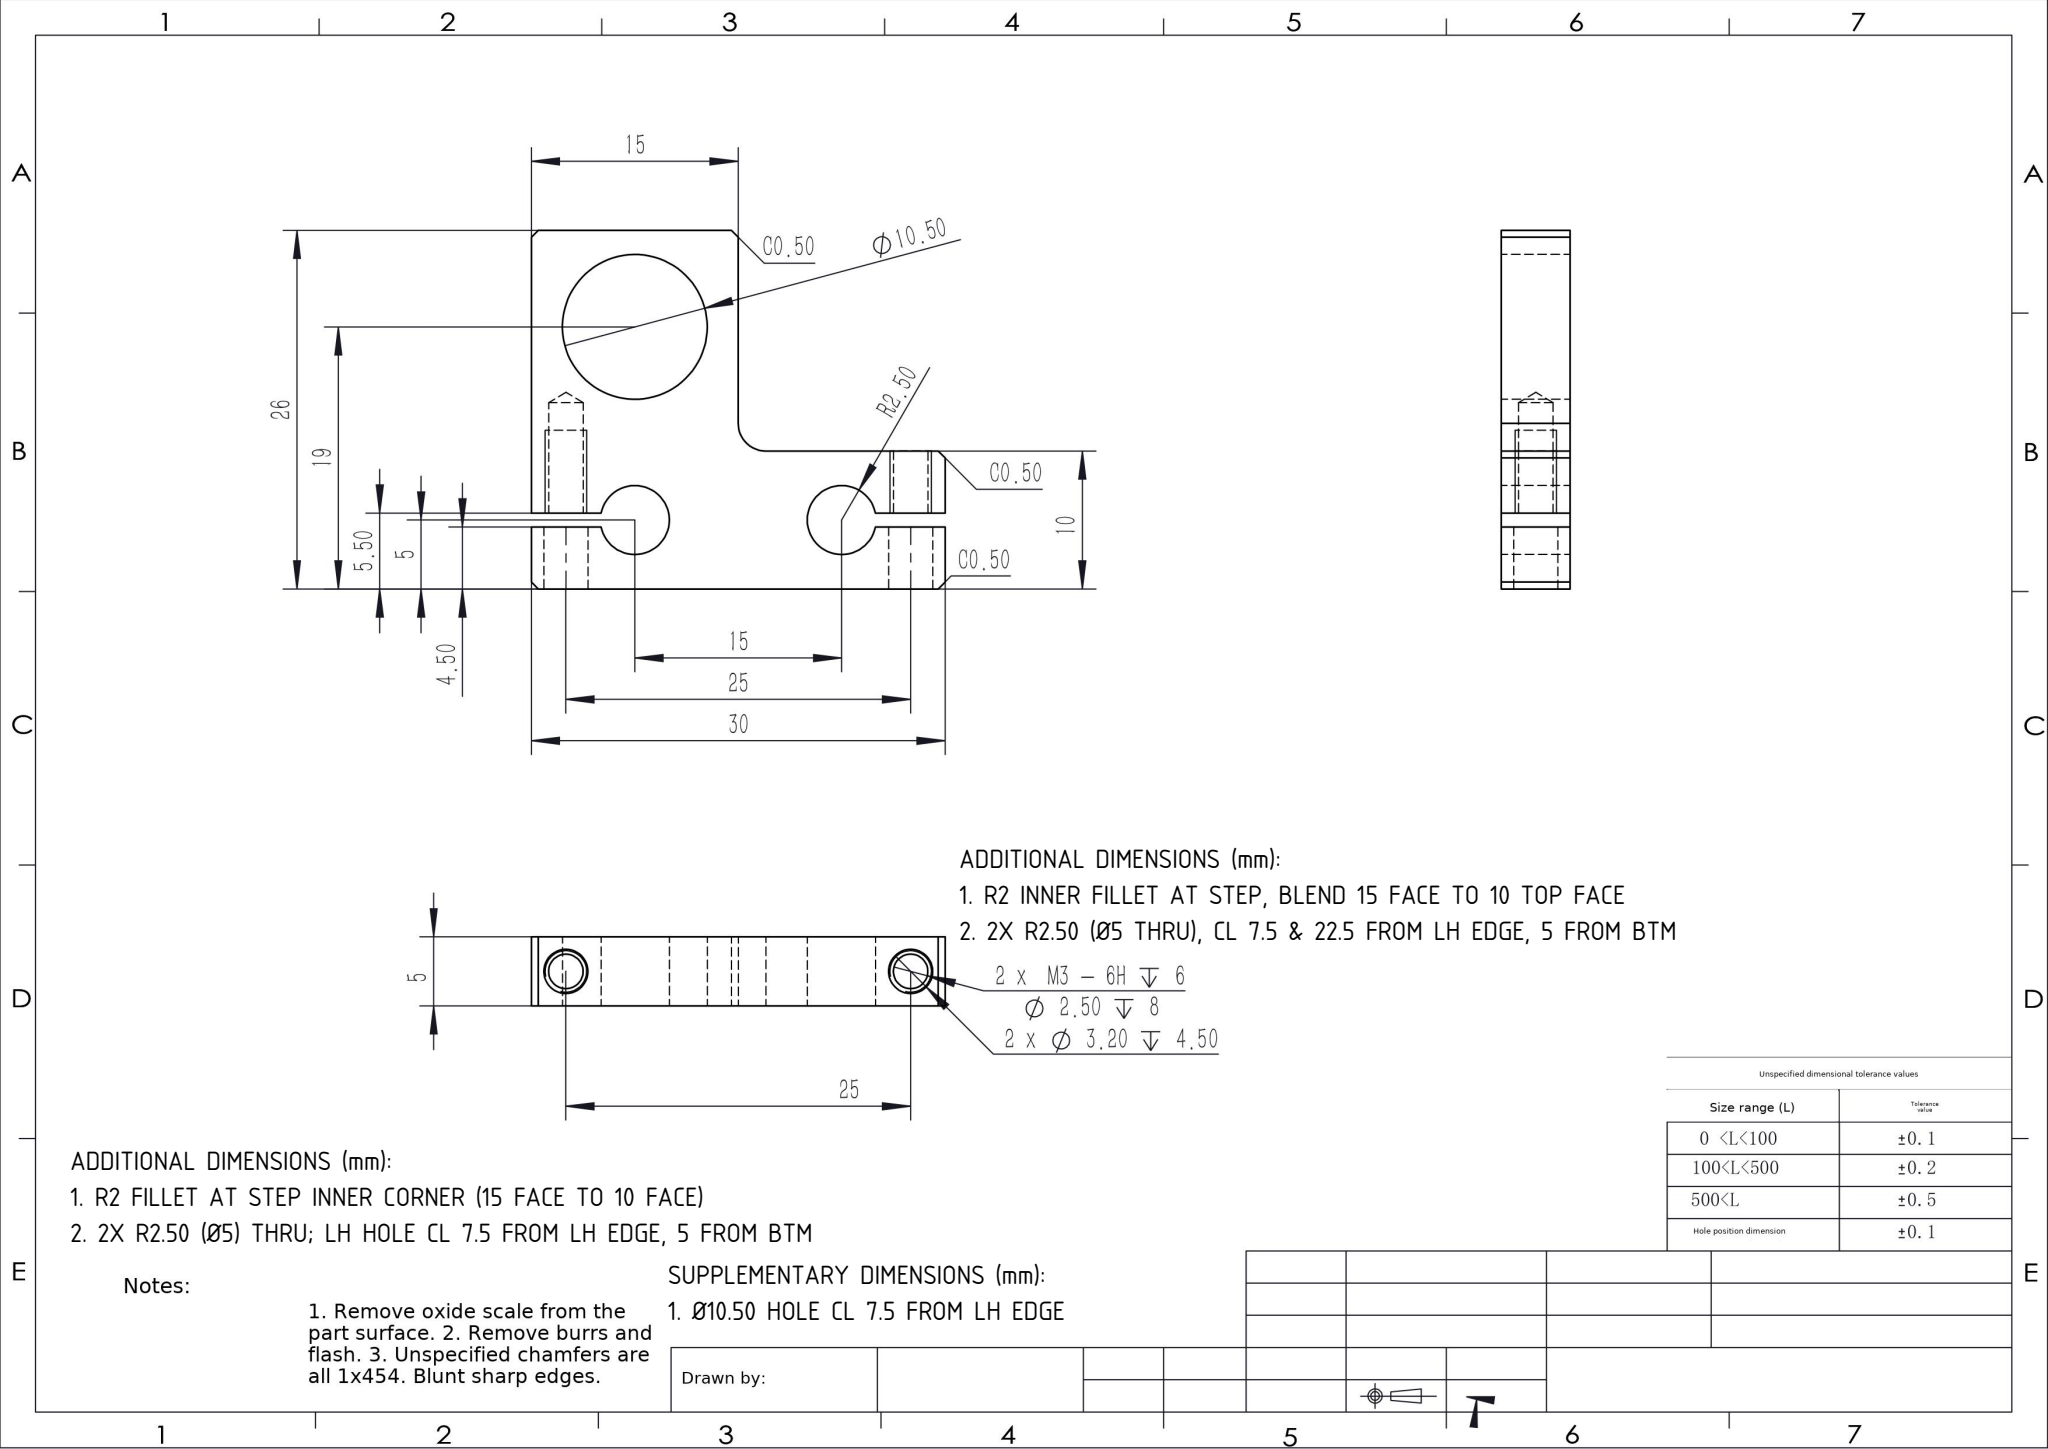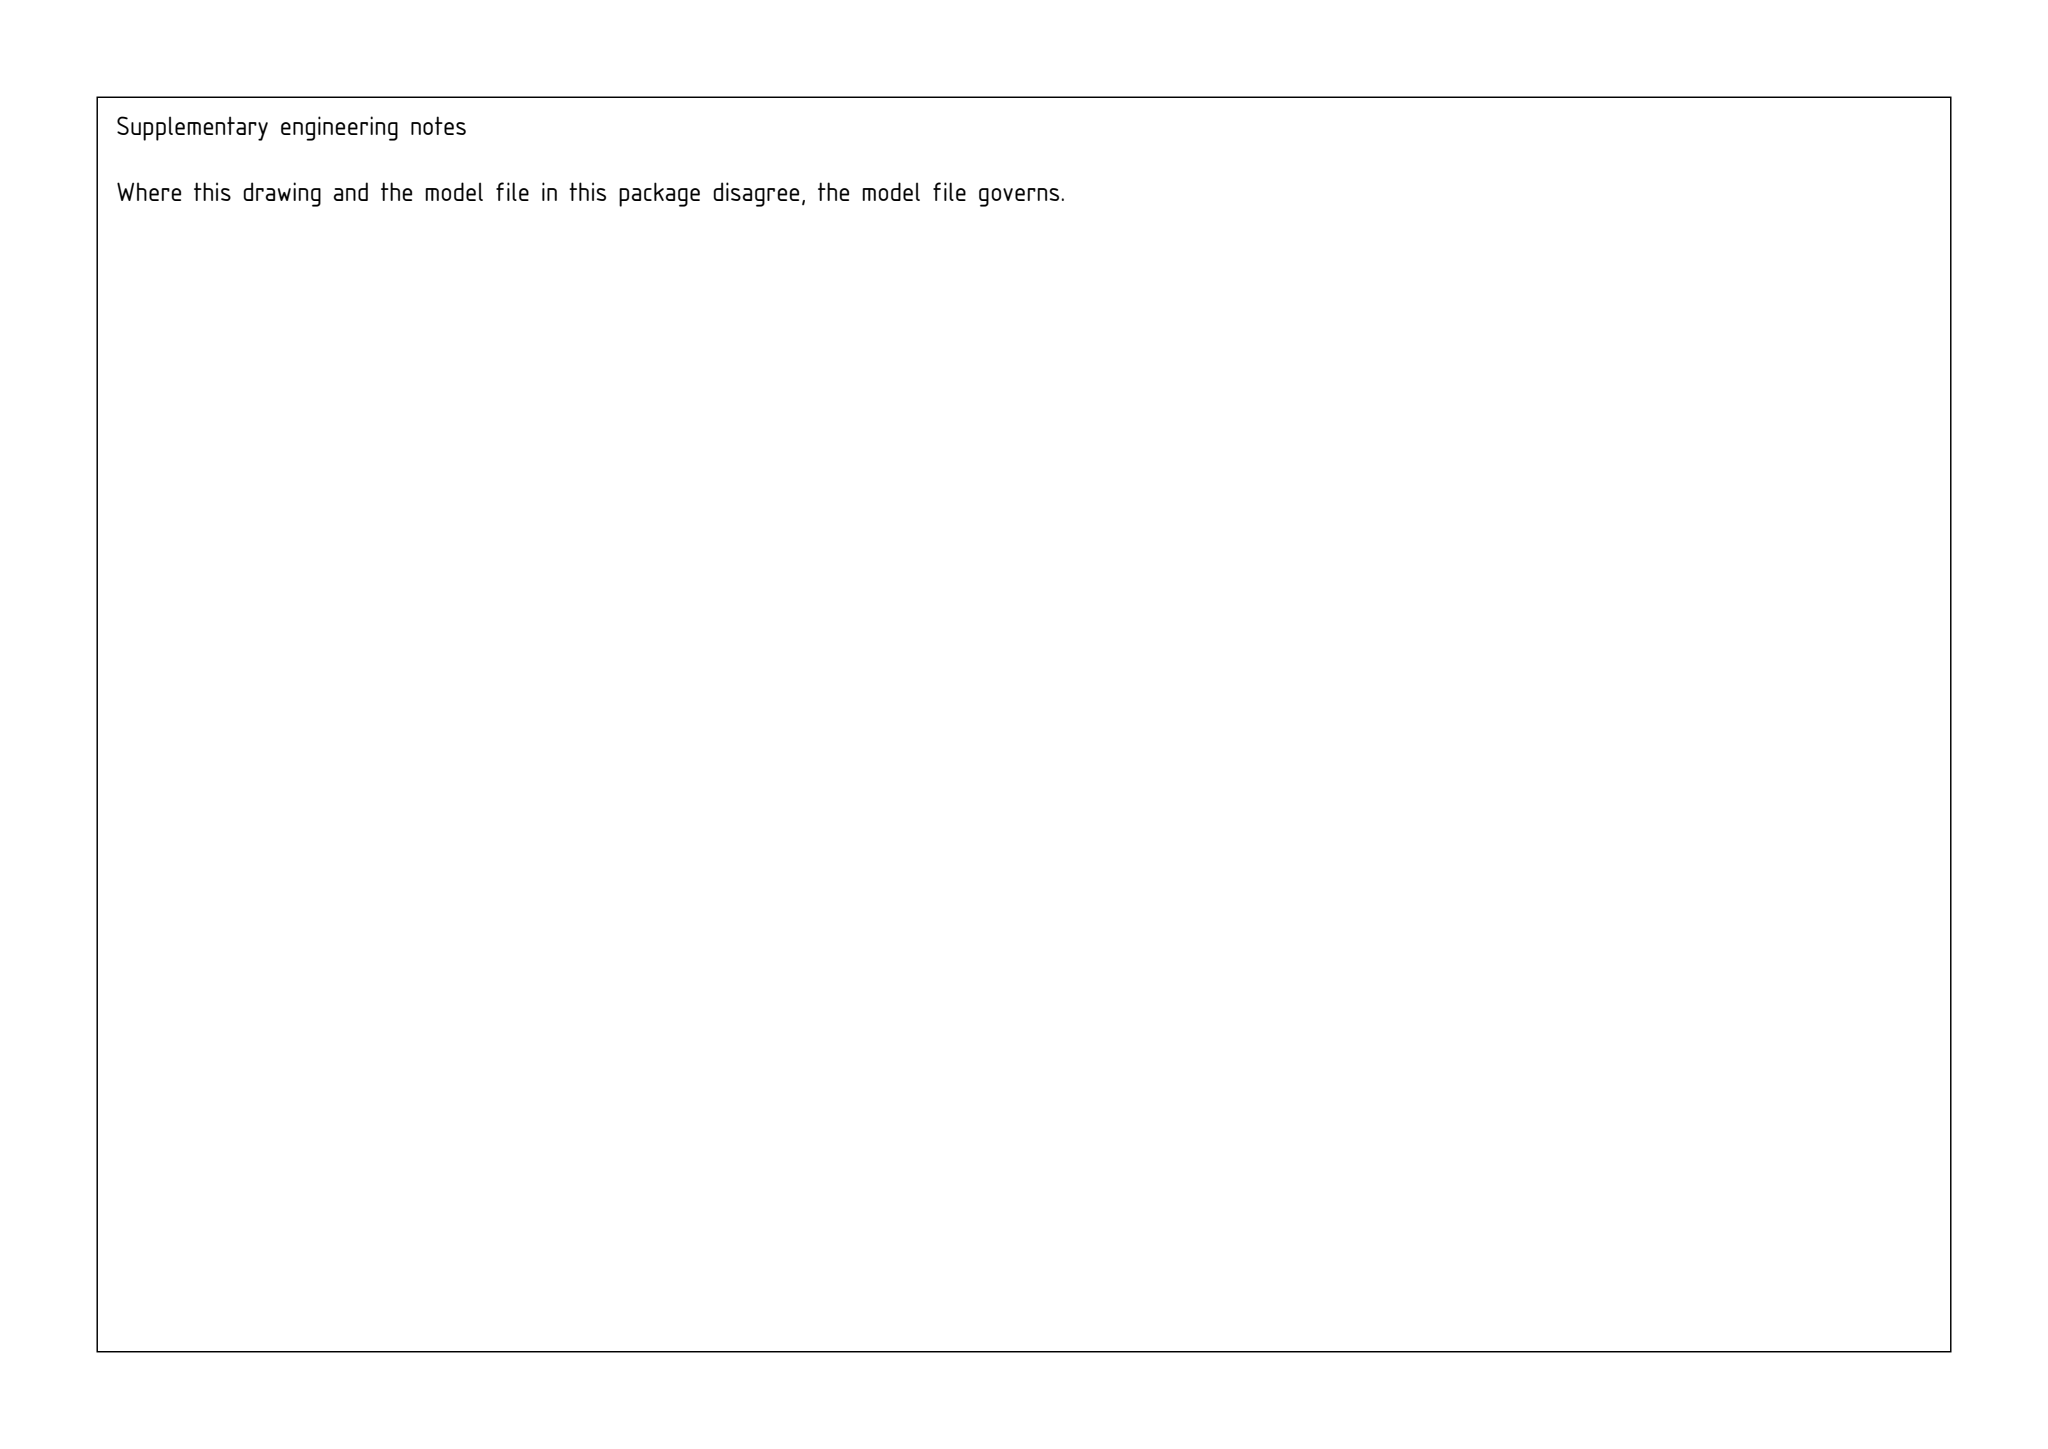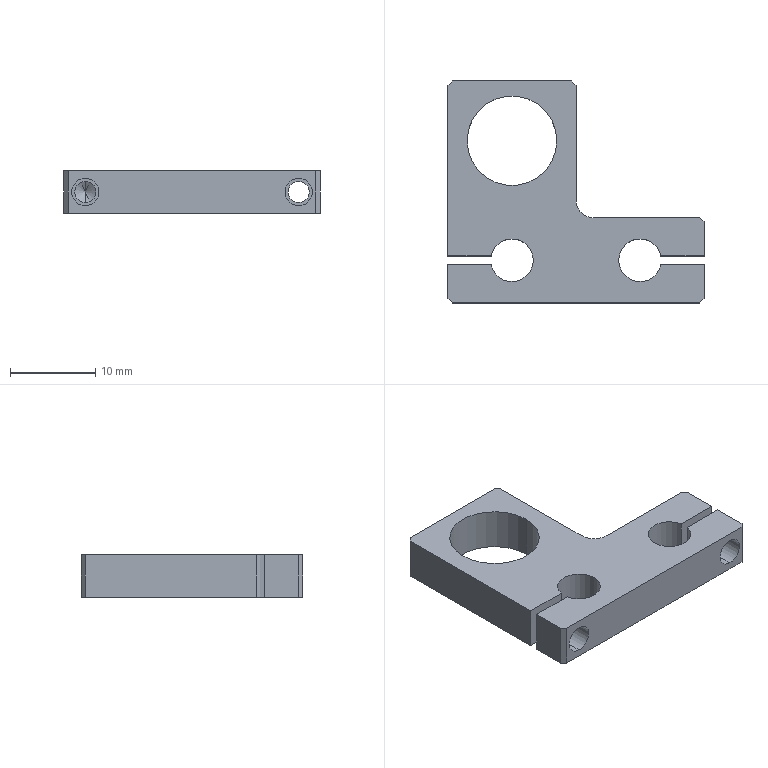Part | SolidWorks | mm | 1 solid | 35 faces | box 30 x 26 x 5 mm | volume 1887 mm3 | plane 19 | cylinder 14 | cone 2 | commonest cylinder face diameters 3.2 x4 2.5 x4 5 x3 10.5 x2 4 x1
build123d program:
from build123d import *

# Parameters (mm, degrees)
SKETCH1_W                  = 30
SKETCH1_H                  = 30
SKETCH1_R                  = 5.249
SKETCH1_R_2                = 2.5
SKETCH1_R_3                = 5.25
BOSS_EXTRUDE1_DEPTH        = 5
SKETCH13_W                 = 15
SKETCH13_H                 = 20
CUT_EXTRUDE4_DEPTH         = 22.794
SKETCH17_W                 = 7.515
SKETCH17_H                 = 1
SKETCH17_W_2               = 10.053
CUT_EXTRUDE5_DEPTH         = 22.794
M3_TAPPED_HOLE1_AT_2_COUNT = 2
M3_TAPPED_HOLE1_AT_2_PITCH = 25
M3_CLEARANCE_HOLE3_D       = 3.2
M3_CLEARANCE_HOLE3_DEPTH   = 4.5
M3_CLEARANCE_HOLE3_TIP     = 0.9614
SKETCH22_W                 = 15
SKETCH22_H                 = 4
CUT_EXTRUDE6_DEPTH         = 22.794
CHAMFER1_SIZE              = 0.5
FILLET1_R                  = 2


with BuildPart() as part:
    # Sketch1 → Boss-Extrude1 (new body)
    with BuildSketch(Plane.XY):
        Rectangle(SKETCH1_W, SKETCH1_H)
        with Locations((7.5, 4)):
            Circle(SKETCH1_R, mode=Mode.SUBTRACT)
        with Locations((-7.5, -10)):
            Circle(SKETCH1_R_2, mode=Mode.SUBTRACT)
        with Locations((-7.5, 4)):
            Circle(SKETCH1_R_3, mode=Mode.SUBTRACT)
        with Locations((7.5, -10)):
            Circle(SKETCH1_R_2, mode=Mode.SUBTRACT)
    extrude(amount=BOSS_EXTRUDE1_DEPTH)

    # Sketch13 → Cut-Extrude4 (cut, through all)
    with BuildSketch(Plane.XY.offset(5)):
        with Locations((7.5, 5)):
            Rectangle(SKETCH13_W, SKETCH13_H)
    extrude(amount=-CUT_EXTRUDE4_DEPTH, mode=Mode.SUBTRACT)

    # Sketch17 → Cut-Extrude5 (cut, through all)
    with BuildSketch(Plane.XY.offset(5)):
        with Locations((13.707, -10)):
            Rectangle(SKETCH17_W, SKETCH17_H)
        with Locations((-14.976, -10)):
            Rectangle(SKETCH17_W_2, SKETCH17_H)
    extrude(amount=-CUT_EXTRUDE5_DEPTH, mode=Mode.SUBTRACT)

    # Sketch18 → M3 Tapped Hole1 (revolve, cut)
    with BuildSketch(Plane(origin=(-12.5, -9.5, 2.5), x_dir=(0, 0, -1), z_dir=(1, 0, 0))):
        Polygon((0, 0), (0, 8.751), (1.25, 8), (1.25, 0), align=None)
    m3_tapped_hole1 = revolve(axis=Axis((-12.5, -15.85, 2.5), (0, 1, 0)), mode=Mode.SUBTRACT)

    # M3 Tapped Hole1 at 2: M3 Tapped Hole1 ×2
    with Locations(*[(i * M3_TAPPED_HOLE1_AT_2_PITCH, 0, 0) for i in range(1, M3_TAPPED_HOLE1_AT_2_COUNT)]):
        add(m3_tapped_hole1, mode=Mode.SUBTRACT)

    # M3 Clearance Hole3
    with Locations(Plane(origin=(0, -15, 0), x_dir=(-1, 0, 0), z_dir=(0, -1, 0))):
        with Locations((12.5, -2.5), (-12.5, -2.5)):
            Hole(M3_CLEARANCE_HOLE3_D / 2, depth=M3_CLEARANCE_HOLE3_DEPTH)
            with Locations((0, 0, -(M3_CLEARANCE_HOLE3_DEPTH + M3_CLEARANCE_HOLE3_TIP / 2))):  # 118° drill point
                Cone(0, M3_CLEARANCE_HOLE3_D / 2, M3_CLEARANCE_HOLE3_TIP, mode=Mode.SUBTRACT)

    # Sketch22 → Cut-Extrude6 (cut, through all)
    with BuildSketch(Plane.XY.offset(5)):
        with Locations((-7.5, 13)):
            Rectangle(SKETCH22_W, SKETCH22_H)
    extrude(amount=-CUT_EXTRUDE6_DEPTH, mode=Mode.SUBTRACT)

    # Chamfer1
    chamfer1_edges = [part.edges().sort_by_distance(p)[0] for p in [
        (-15, 11, 2.5),
        (0, 11, 2.5),
        (15, -5, 2.5),
        (15, -15, 2.5),
        (-15, -15, 2.5),
    ]]
    chamfer(chamfer1_edges, length=CHAMFER1_SIZE)

    # Fillet1
    fillet1_edges = [part.edges().sort_by_distance(p)[0] for p in [
        (0, -5, 2.5),
    ]]
    fillet(fillet1_edges, radius=FILLET1_R)


solid = part.part